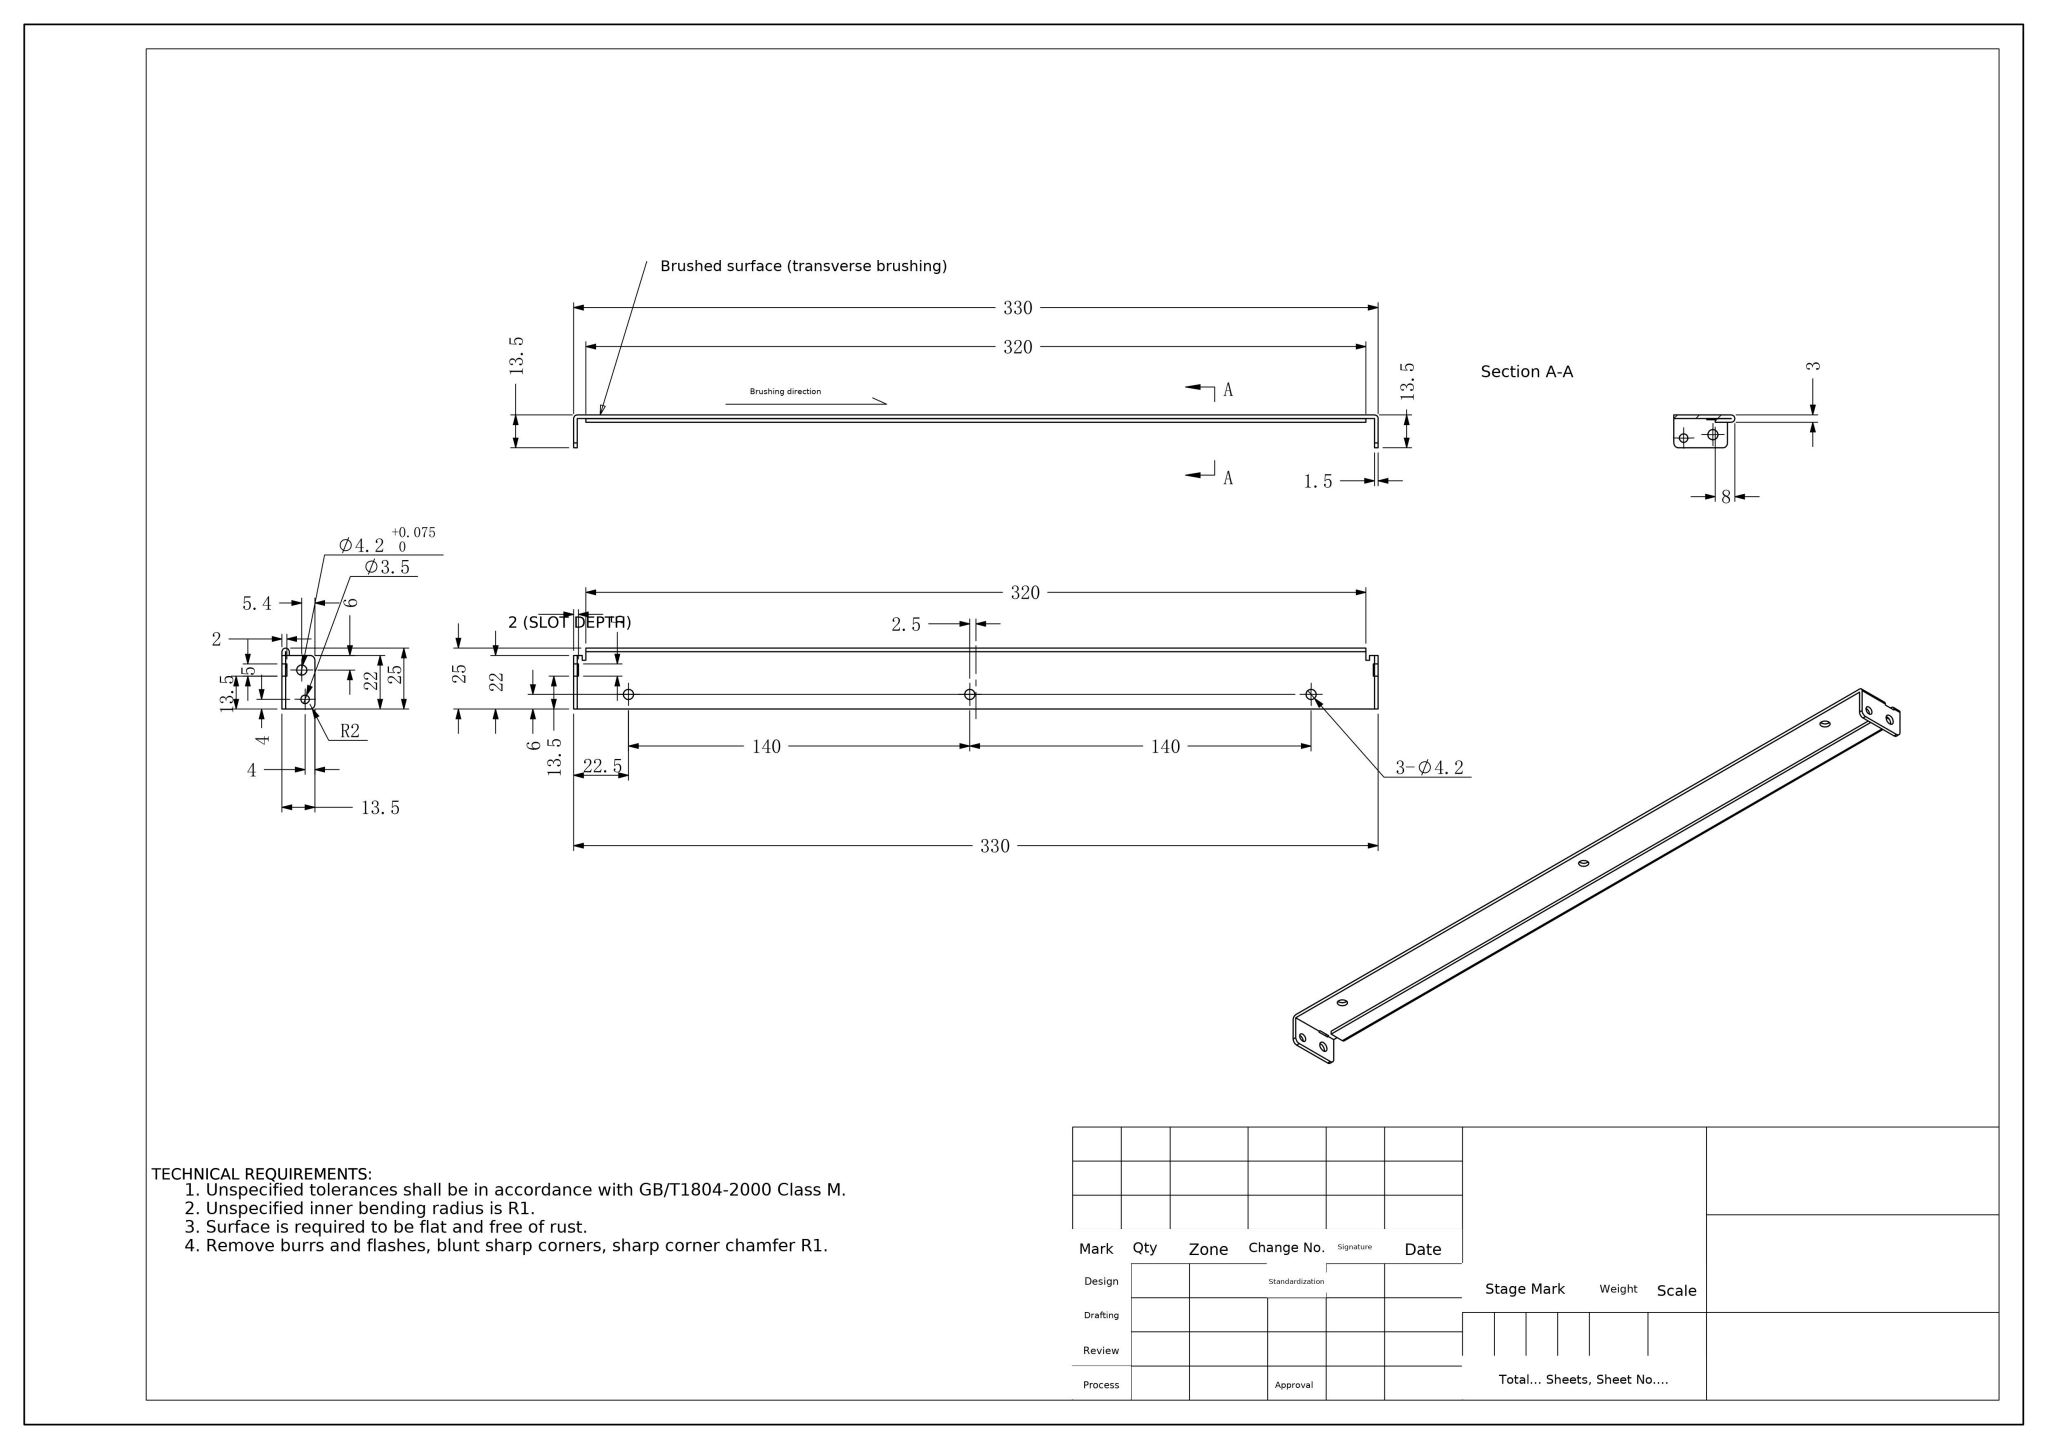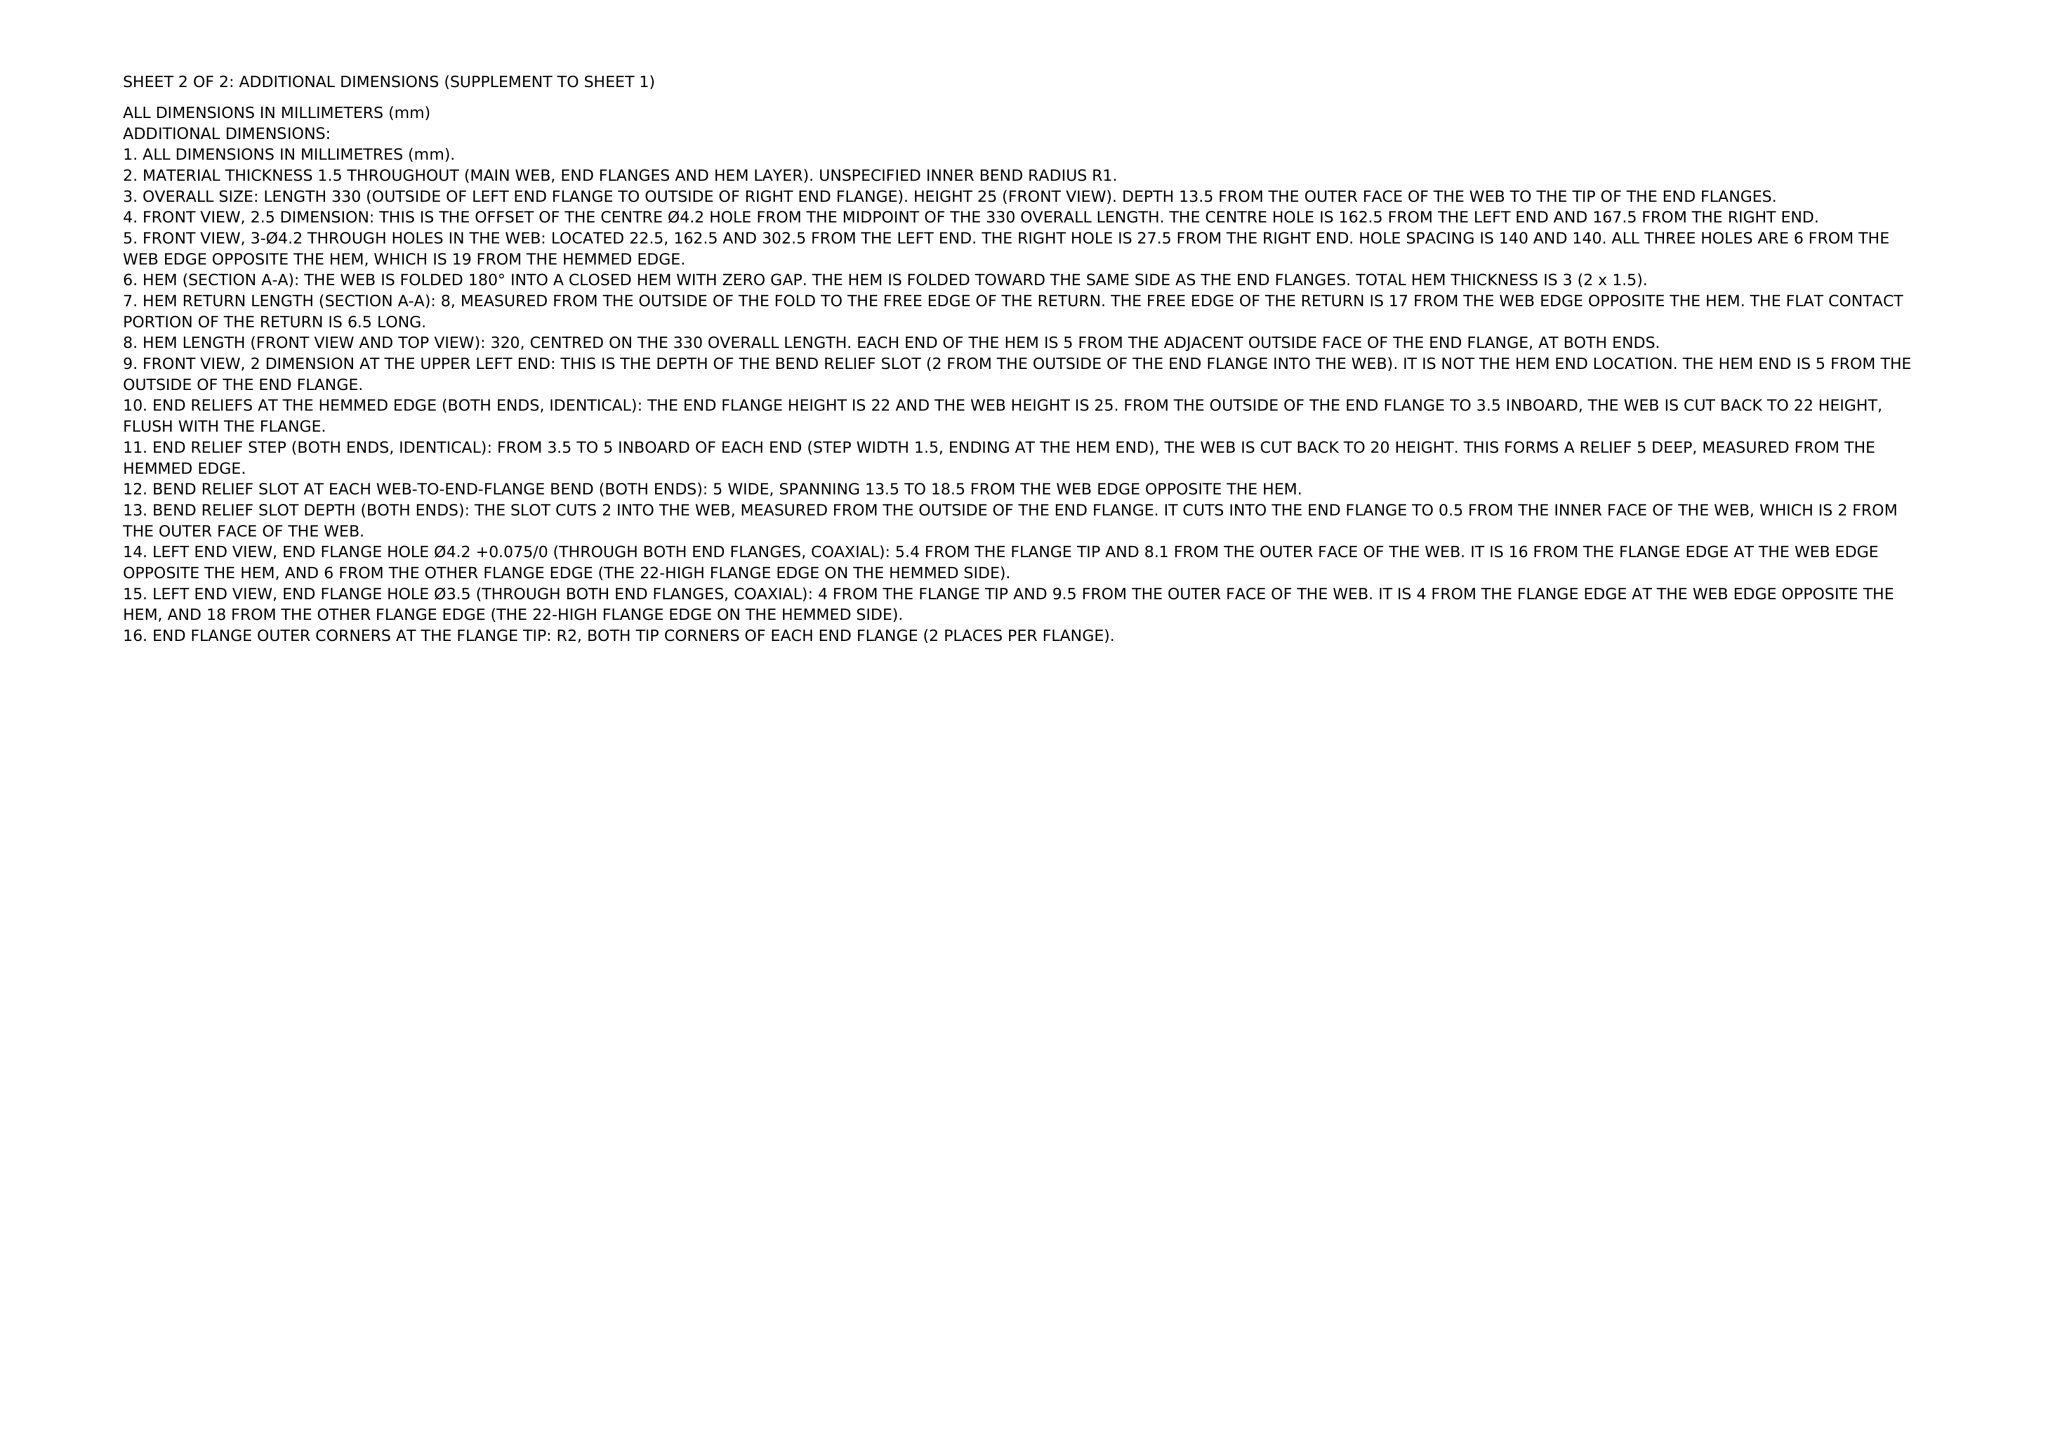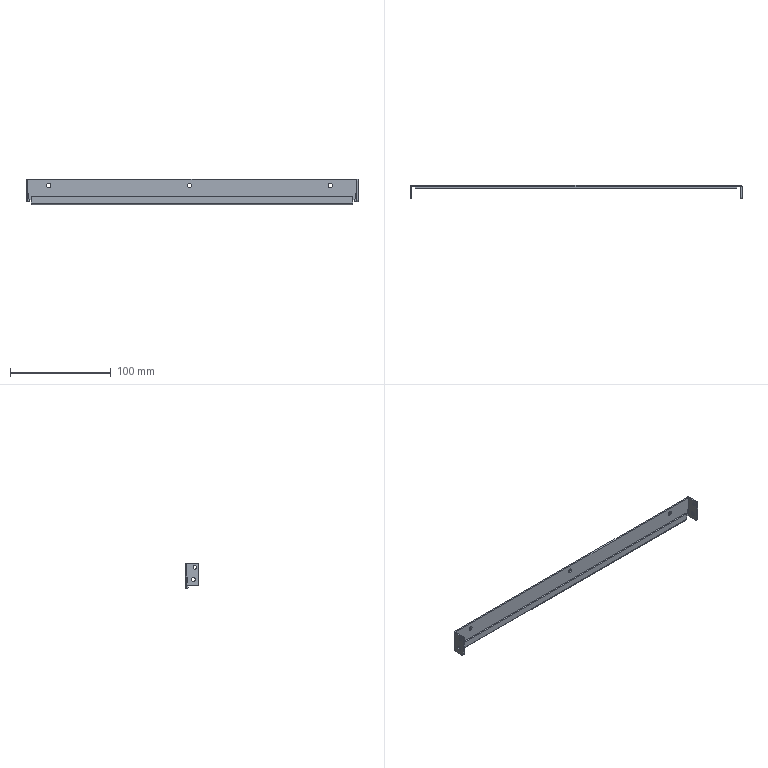Part | NX | mm | 1 solid | 60 faces | box 330 x 13.5 x 25 mm | volume 16456 mm3 | cylinder 30 | plane 30 | commonest cylinder face diameters 4.2 x10 3.004 x6 0.004 x6 3.5 x4 4 x4